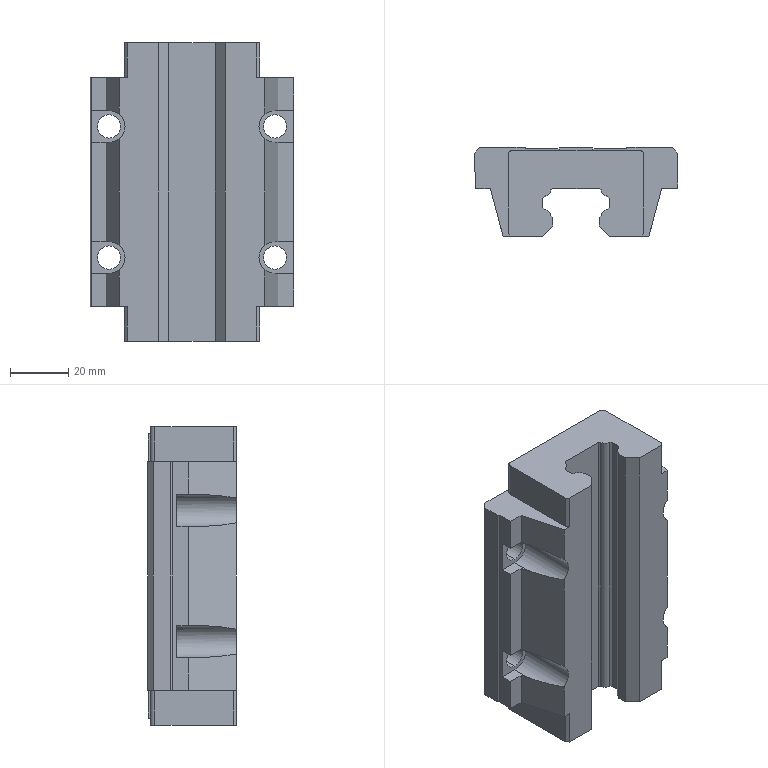Component | SolidWorks | HG_BLOCK_HGWHC_ANY-1 | 1 solid | 98 faces | volume 140366 mm3 | plane 78 | cylinder 20 | commonest cylinder face diameters 8 x8 4.6 x4 3 x4 11 x4